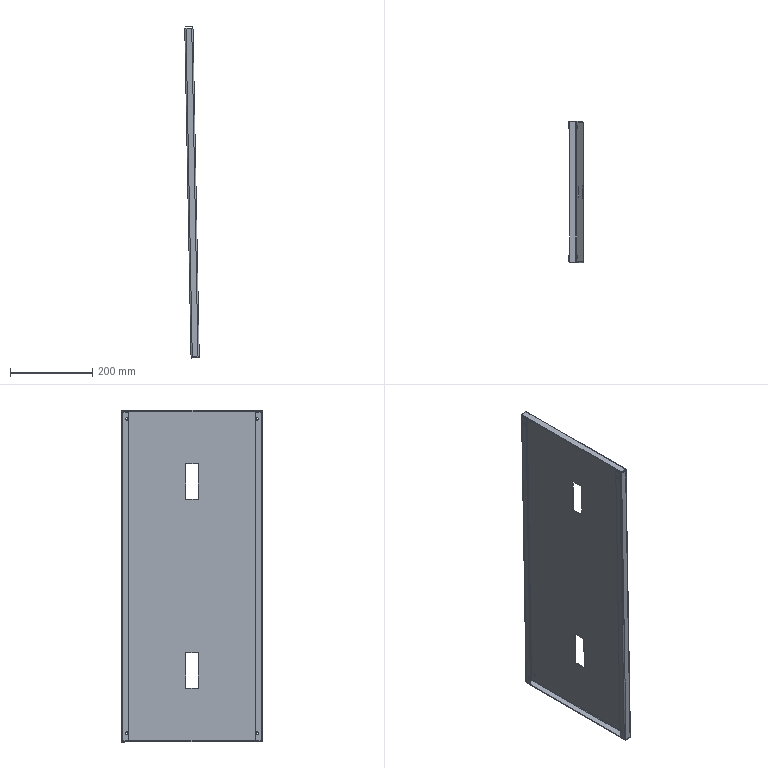Component | SolidWorks | 05FrameEndPlate4-1 | 1 solid | 88 faces | volume 663885 mm3 | plane 60 | cylinder 28 | commonest cylinder face diameters 7 x16 6 x6 2 x6 | material A3 Steel